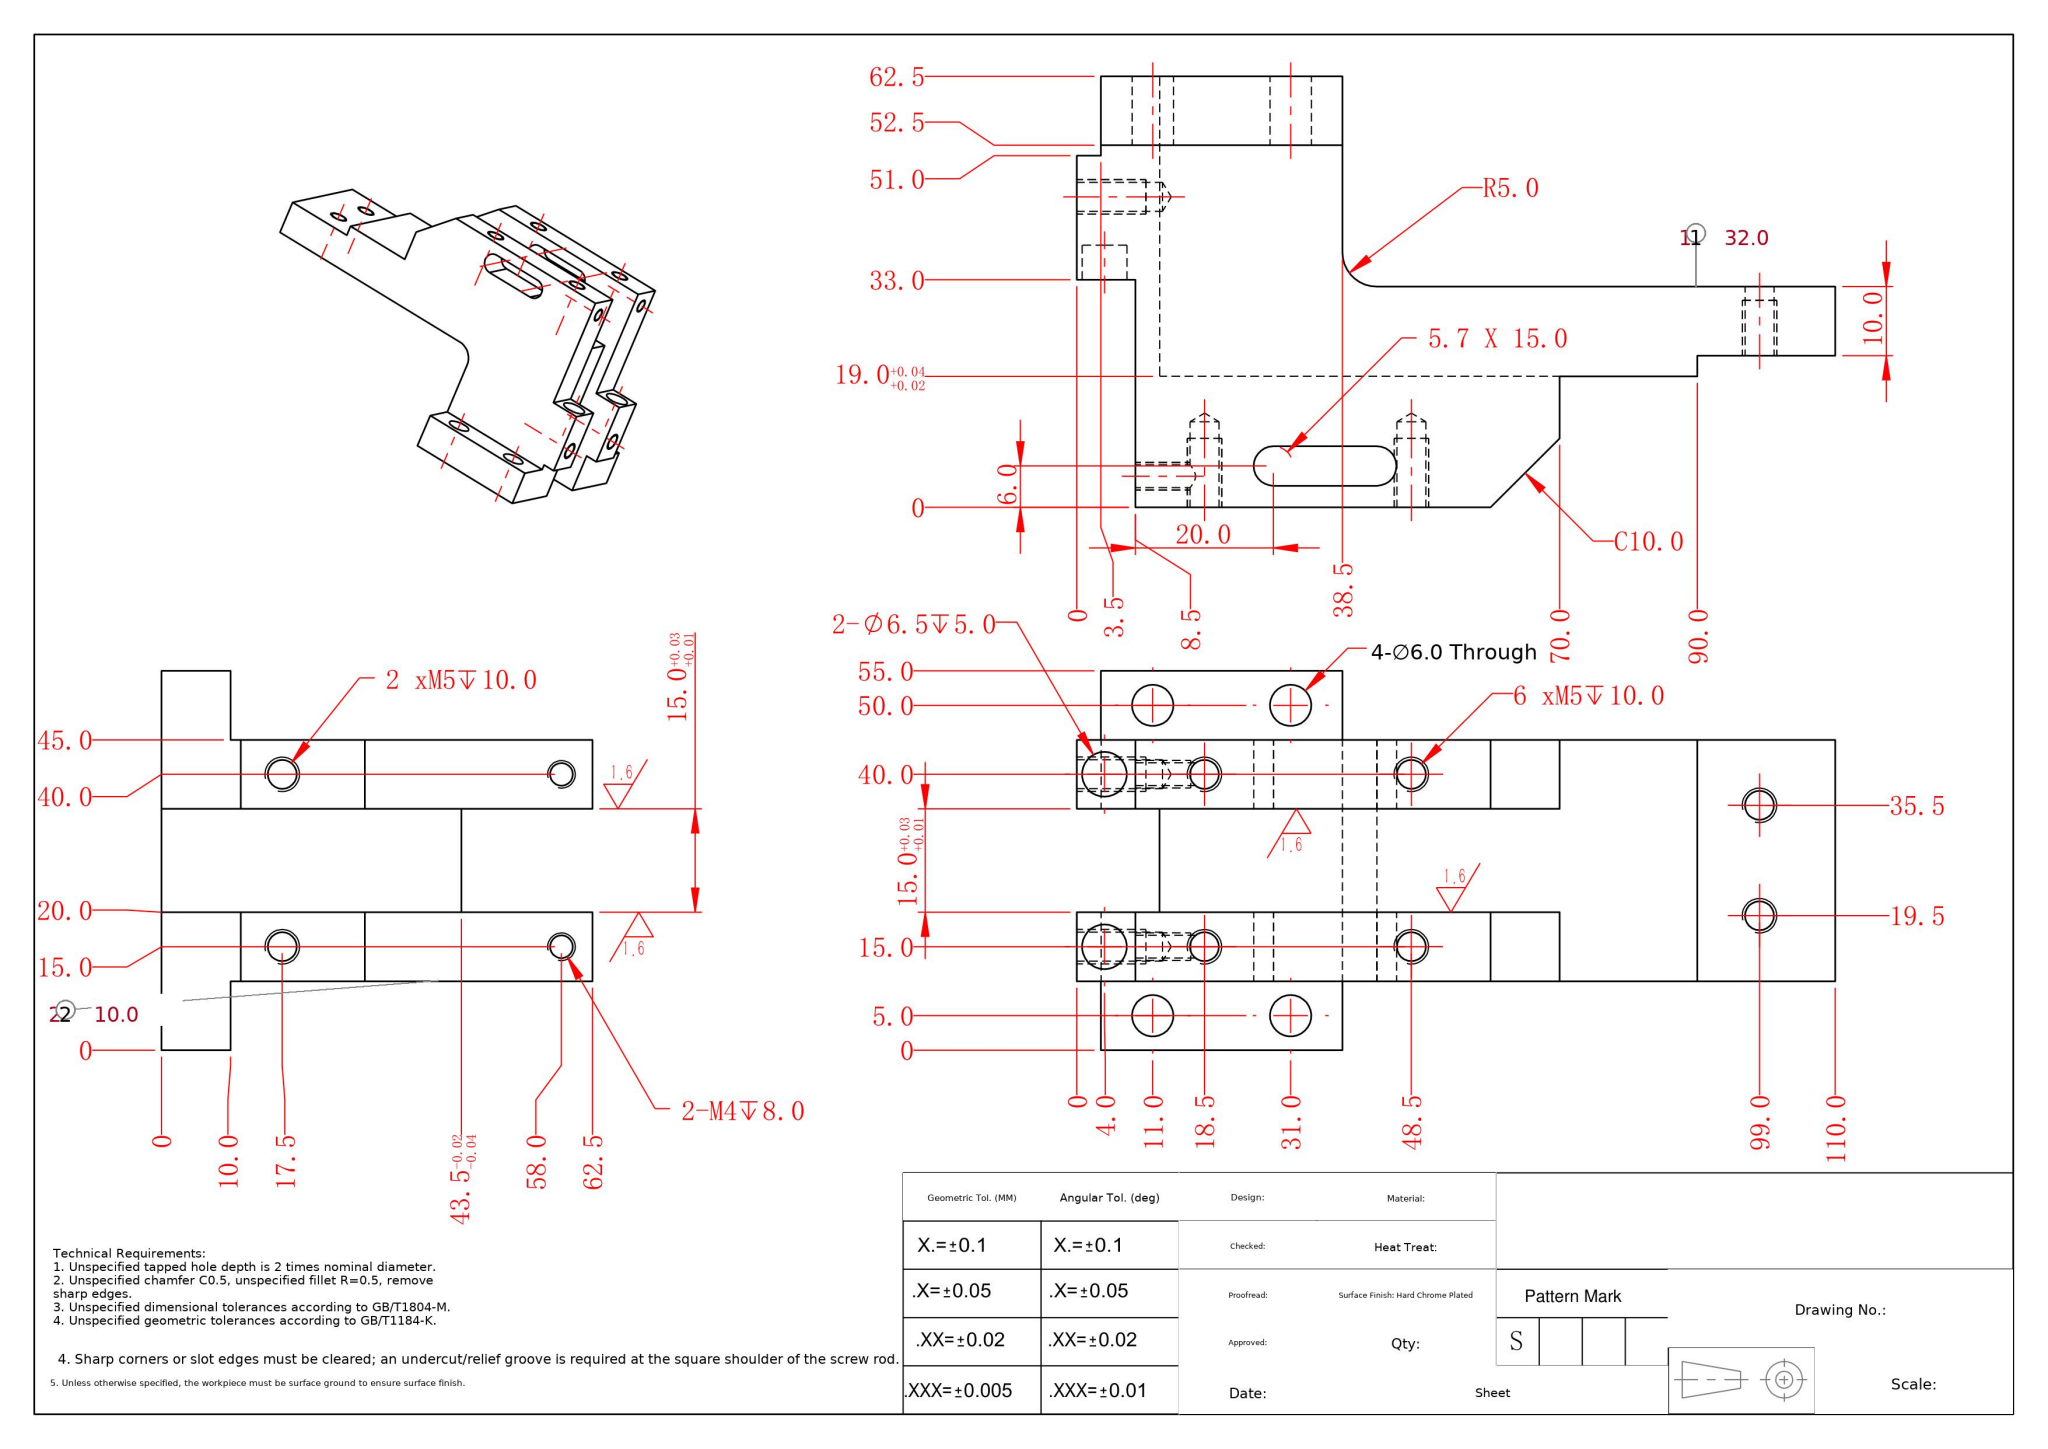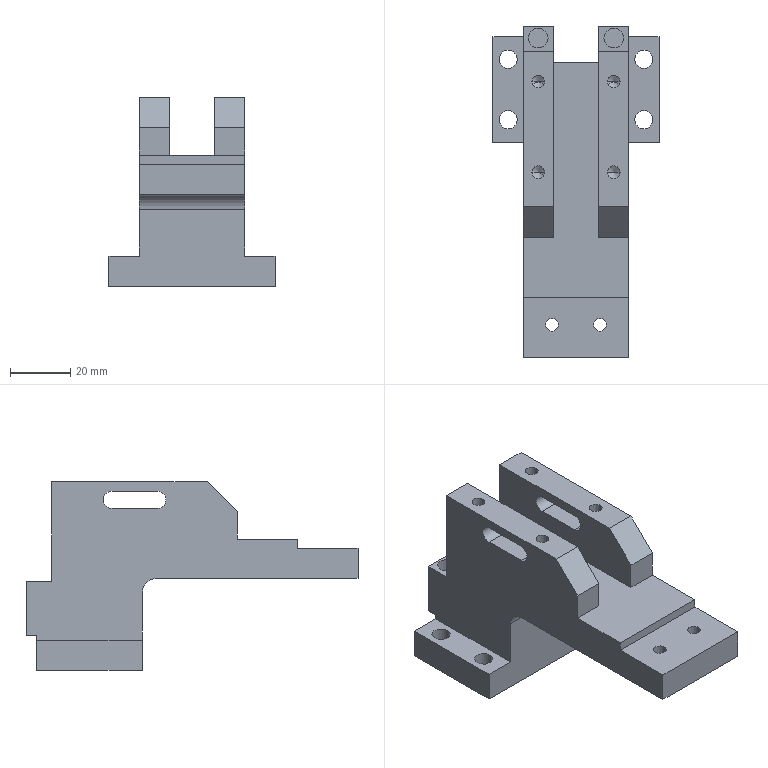Part | SolidWorks | mm | 1 solid | 89 faces | box 55 x 110 x 62.5 mm | volume 102416 mm3 | cylinder 39 | plane 38 | cone 12 | commonest cylinder face diameters 4.2 x16 6 x8 5.724 x6 3.3 x4 6.5 x4 10 x1
build123d program:
from build123d import *

# Parameters (mm, degrees)
SKETCH1_W             = 35
SKETCH1_H             = 110
BOSS_EXTRUDE1_DEPTH   = 62.5
SKETCH2_W             = 15
SKETCH2_H             = 110
CUT_EXTRUDE1_DEPTH    = 19
SKETCH3_W             = 15
SKETCH3_H             = 43.5
CUT_EXTRUDE2_DEPTH    = 12
SKETCH4_W             = 10
SKETCH4_H             = 35
BOSS_EXTRUDE2_DEPTH   = 10
SKETCH5_W             = 35
SKETCH5_H             = 33
CUT_EXTRUDE3_DEPTH    = 8.5
SKETCH6_R             = 3.25
CUT_EXTRUDE4_DEPTH    = 5
SKETCH8_W             = 22
SKETCH8_H             = 20
CUT_EXTRUDE6_DEPTH    = 95.637
SKETCH9_R             = 3
CUT_EXTRUDE7_DEPTH    = 81.855
SKETCH10_W            = 30.5
SKETCH10_H            = 71.5
CUT_EXTRUDE8_DEPTH    = 95.637
FILLET1_R             = 5
M5_TAPPED_HOLE1_D     = 4.2
M5_TAPPED_HOLE1_DEPTH = 12.4
M5_TAPPED_HOLE1_TIP   = 1.262
M4_TAPPED_HOLE1_D     = 3.3
M4_TAPPED_HOLE1_DEPTH = 10.1
M4_TAPPED_HOLE1_TIP   = 0.9914
M5_TAPPED_HOLE2_D     = 4.2
M5_TAPPED_HOLE2_DEPTH = 12.4
M5_TAPPED_HOLE2_TIP   = 1.262
M5_TAPPED_HOLE3_D     = 4.2
M5_TAPPED_HOLE3_DEPTH = 12.4
M5_TAPPED_HOLE3_TIP   = 1.262
SKETCH19_W            = 11.5
SKETCH19_H            = 3.5
CUT_EXTRUDE9_DEPTH    = 95.637
SKETCH20_W            = 19
SKETCH20_H            = 20
CUT_EXTRUDE10_DEPTH   = 95.637
CHAMFER1_SIZE         = 10
CUT_EXTRUDE11_DEPTH   = 95.637


with BuildPart() as part:
    # Sketch1 → Boss-Extrude1 (new body)
    with BuildSketch(Plane.XY):
        Rectangle(SKETCH1_W, SKETCH1_H)
    extrude(amount=BOSS_EXTRUDE1_DEPTH)

    # Sketch2 → Cut-Extrude1 (cut)
    with BuildSketch(Plane.XY.offset(62.5)):
        Rectangle(SKETCH2_W, SKETCH2_H)
    extrude(amount=-CUT_EXTRUDE1_DEPTH, mode=Mode.SUBTRACT)

    # Sketch3 → Cut-Extrude2 (cut)
    with BuildSketch(Plane(origin=(0, 55, 0), x_dir=(1, 0, 0), z_dir=(0, 1, 0))):
        with Locations((0, -21.75)):
            Rectangle(SKETCH3_W, SKETCH3_H)
    extrude(amount=-CUT_EXTRUDE2_DEPTH, mode=Mode.SUBTRACT)

    # Sketch4 → Boss-Extrude2 (add)
    with BuildSketch(Plane(origin=(0, 0, 0), x_dir=(-1, 0, 0), z_dir=(0, 0, -1))):
        with Locations((22.5, 34)):
            Rectangle(SKETCH4_W, SKETCH4_H)
        with Locations((-22.5, 34)):
            Rectangle(SKETCH4_W, SKETCH4_H)
    extrude(amount=-BOSS_EXTRUDE2_DEPTH)

    # Sketch5 → Cut-Extrude3 (cut)
    with BuildSketch(Plane(origin=(0, 55, 0), x_dir=(1, 0, 0), z_dir=(0, 1, 0))):
        with Locations((0, -46)):
            Rectangle(SKETCH5_W, SKETCH5_H)
    extrude(amount=-CUT_EXTRUDE3_DEPTH, mode=Mode.SUBTRACT)

    # Sketch6 → Cut-Extrude4 (cut)
    with BuildSketch(Plane.XY.offset(29.5)):
        with Locations((-12.5, 51)):
            Circle(SKETCH6_R)
        with Locations((12.5, 51)):
            Circle(SKETCH6_R)
    extrude(amount=-CUT_EXTRUDE4_DEPTH, mode=Mode.SUBTRACT)

    # Sketch8 → Cut-Extrude6 (cut, through all)
    with BuildSketch(Plane.ZY.offset(17.5)):
        with Locations((51.5, -45)):
            Rectangle(SKETCH8_W, SKETCH8_H)
    extrude(amount=-CUT_EXTRUDE6_DEPTH, mode=Mode.SUBTRACT)

    # Sketch9 → Cut-Extrude7 (cut, through all)
    with BuildSketch(Plane.XY.offset(10)):
        with Locations((22.5, 44)):
            Circle(SKETCH9_R)
        with Locations((22.5, 24)):
            Circle(SKETCH9_R)
        with Locations((-22.5, 44)):
            Circle(SKETCH9_R)
        with Locations((-22.5, 24)):
            Circle(SKETCH9_R)
    extrude(amount=-CUT_EXTRUDE7_DEPTH, mode=Mode.SUBTRACT)

    # Sketch10 → Cut-Extrude8 (cut, through all)
    with BuildSketch(Plane.ZY.offset(17.5)):
        with Locations((15.25, -19.25)):
            Rectangle(SKETCH10_W, SKETCH10_H)
    extrude(amount=-CUT_EXTRUDE8_DEPTH, mode=Mode.SUBTRACT)

    # Fillet1
    fillet1_edges = [part.edges().sort_by_distance(p)[0] for p in [
        (0, 16.5, 30.5),
    ]]
    fillet(fillet1_edges, radius=FILLET1_R)

    # M5 Tapped Hole1
    with Locations(Plane.XY.offset(62.5)):
        with Locations((-12.5, 36.5), (12.5, 36.5), (12.5, 6.5), (-12.5, 6.5)):
            Hole(M5_TAPPED_HOLE1_D / 2, depth=M5_TAPPED_HOLE1_DEPTH)
            with Locations((0, 0, -(M5_TAPPED_HOLE1_DEPTH + M5_TAPPED_HOLE1_TIP / 2))):  # 118° drill point
                Cone(0, M5_TAPPED_HOLE1_D / 2, M5_TAPPED_HOLE1_TIP, mode=Mode.SUBTRACT)

    # M4 Tapped Hole1
    with Locations(Plane(origin=(0, 46.5, 0), x_dir=(1, 0, 0), z_dir=(0, 1, 0))):
        with Locations((-12.5, -58), (12.5, -58)):
            Hole(M4_TAPPED_HOLE1_D / 2, depth=M4_TAPPED_HOLE1_DEPTH)
            with Locations((0, 0, -(M4_TAPPED_HOLE1_DEPTH + M4_TAPPED_HOLE1_TIP / 2))):  # 118° drill point
                Cone(0, M4_TAPPED_HOLE1_D / 2, M4_TAPPED_HOLE1_TIP, mode=Mode.SUBTRACT)

    # M5 Tapped Hole2
    with Locations(Plane(origin=(0, 55, 0), x_dir=(1, 0, 0), z_dir=(0, 1, 0))):
        with Locations((-12.5, -17.5), (12.5, -17.5)):
            Hole(M5_TAPPED_HOLE2_D / 2, depth=M5_TAPPED_HOLE2_DEPTH)
            with Locations((0, 0, -(M5_TAPPED_HOLE2_DEPTH + M5_TAPPED_HOLE2_TIP / 2))):  # 118° drill point
                Cone(0, M5_TAPPED_HOLE2_D / 2, M5_TAPPED_HOLE2_TIP, mode=Mode.SUBTRACT)

    # M5 Tapped Hole3
    with Locations(Plane.XY.offset(40.5)):
        with Locations((-8, -44), (8, -44)):
            Hole(M5_TAPPED_HOLE3_D / 2, depth=M5_TAPPED_HOLE3_DEPTH)
            with Locations((0, 0, -(M5_TAPPED_HOLE3_DEPTH + M5_TAPPED_HOLE3_TIP / 2))):  # 118° drill point
                Cone(0, M5_TAPPED_HOLE3_D / 2, M5_TAPPED_HOLE3_TIP, mode=Mode.SUBTRACT)

    # Sketch19 → Cut-Extrude9 (cut, through all)
    with BuildSketch(Plane.ZY.offset(17.5)):
        with Locations((5.75, 53.25)):
            Rectangle(SKETCH19_W, SKETCH19_H)
    extrude(amount=-CUT_EXTRUDE9_DEPTH, mode=Mode.SUBTRACT)

    # Sketch20 → Cut-Extrude10 (cut, through all)
    with BuildSketch(Plane(origin=(17.5, 0, 0), x_dir=(0, 0, -1), z_dir=(1, 0, 0))):
        with Locations((-53, -25)):
            Rectangle(SKETCH20_W, SKETCH20_H)
    extrude(amount=-CUT_EXTRUDE10_DEPTH, mode=Mode.SUBTRACT)

    # Chamfer1
    chamfer1_edges = [part.edges().sort_by_distance(p)[0] for p in [
        (-12.5, -15, 62.5),
        (12.5, -15, 62.5),
    ]]
    chamfer(chamfer1_edges, length=CHAMFER1_SIZE)

    # Sketch21 → Cut-Extrude11 (cut, through all)
    with BuildSketch(Plane.ZY.offset(17.5)):
        with BuildLine():
            Line((59.362, 26.5), (59.362, 11.5))
            ThreePointArc((59.362, 11.5), (56.5, 8.638), (53.638, 11.5))
            Line((53.638, 11.5), (53.638, 26.5))
            ThreePointArc((53.638, 26.5), (56.5, 29.362), (59.362, 26.5))
        make_face()
    extrude(amount=-CUT_EXTRUDE11_DEPTH, mode=Mode.SUBTRACT)


solid = part.part